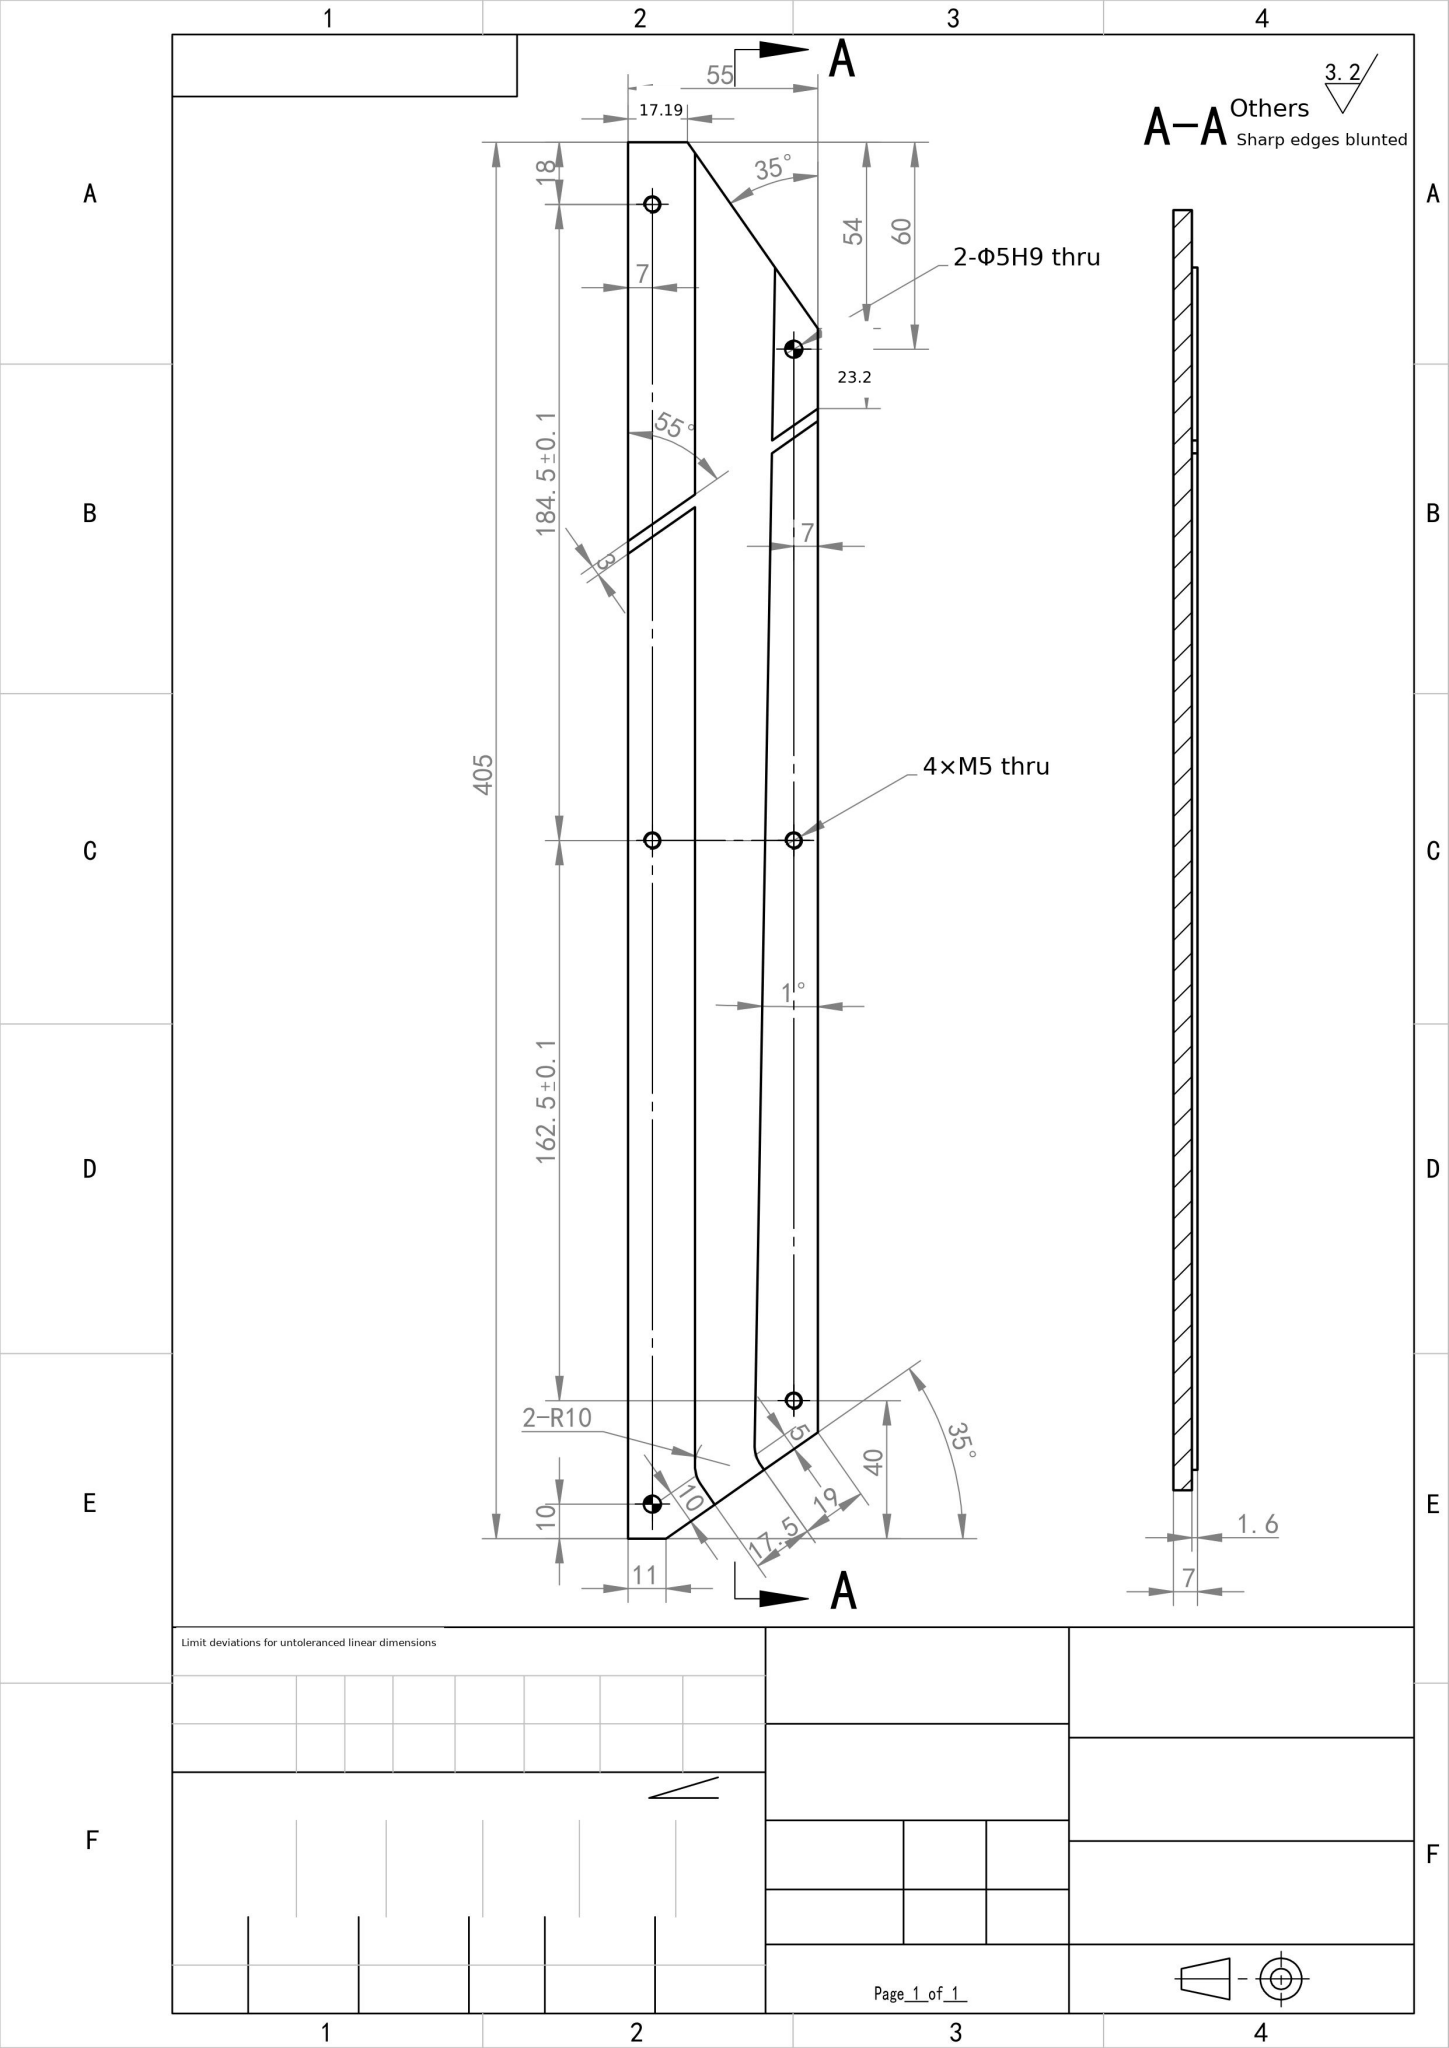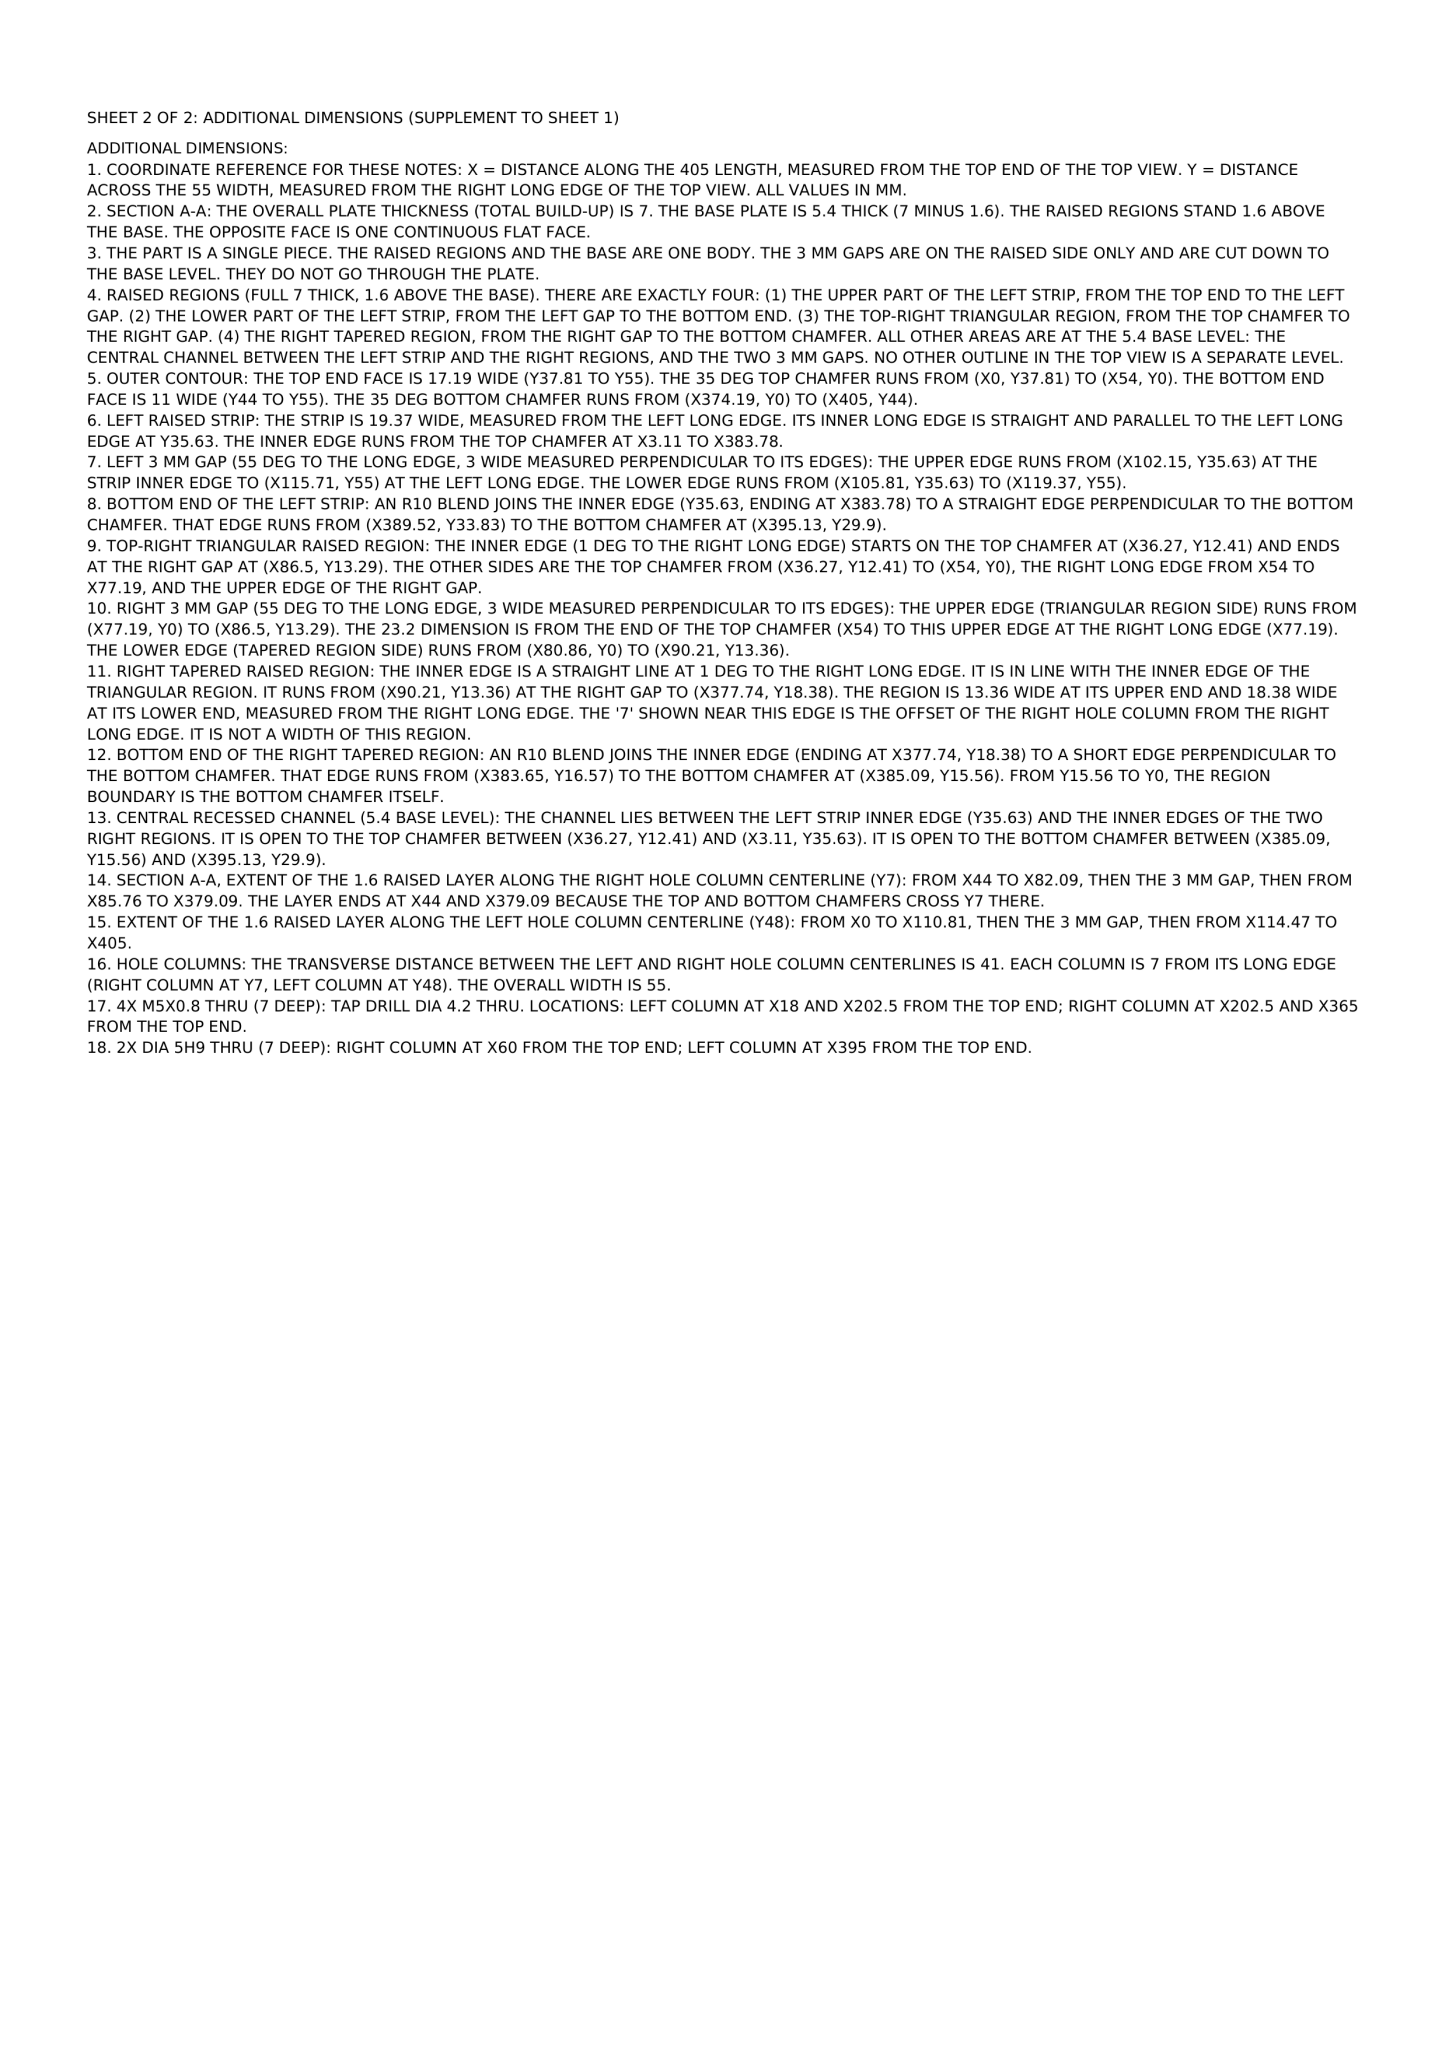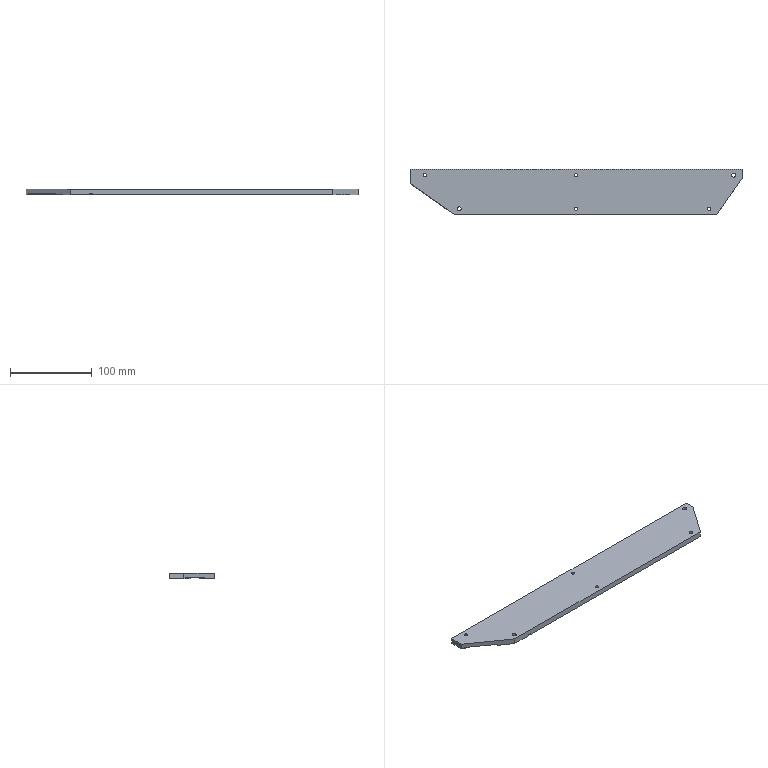Part | NX | mm | 1 solid | 36 faces | box 405 x 55 x 7 mm | volume 131124 mm3 | plane 22 | cylinder 14 | commonest cylinder face diameters 4.2 x8 5 x4 20 x2